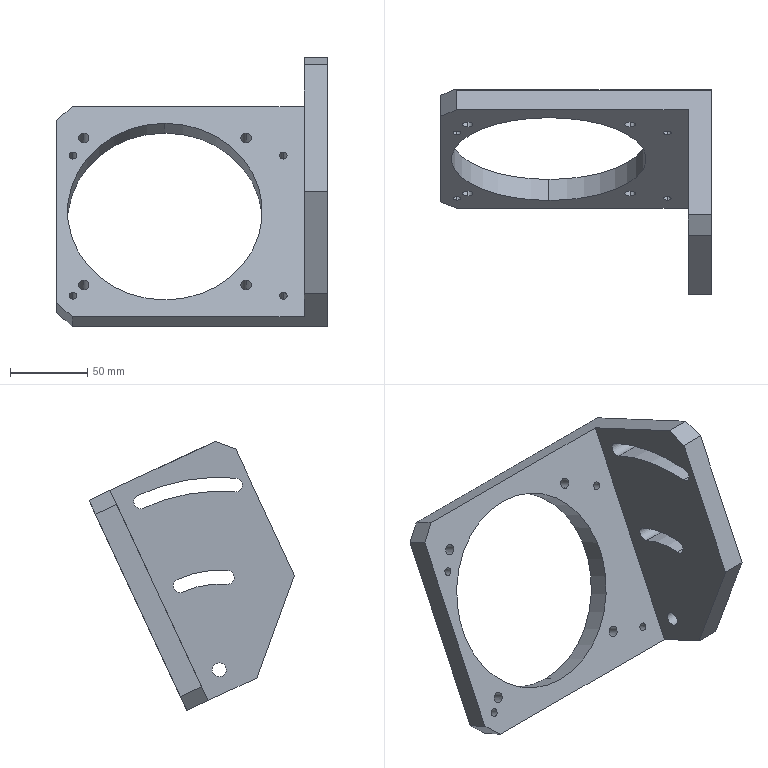Component | SolidWorks | 17081801-804-004A-1 | 1 solid | 41 faces | box 175 x 132.47 x 173.98 mm | volume 357939 mm3 | cylinder 28 | plane 13 | commonest cylinder face diameters 5 x8 6.8 x8 9 x6 126 x2 111 x1 129 x1 231 x1 249 x1 | material AL6061
build123d program:
from build123d import *

# Parameters (mm, degrees)
BOSS_EXTRUDE2_DEPTH   = 75
SKETCH17_R            = 63
CUT_EXTRUDE2_DEPTH    = 197.087
M8_TAPPED_HOLE1_D     = 6.8
M8_TAPPED_HOLE1_DEPTH = 19.75
M8_TAPPED_HOLE1_TIP   = 2.043
M8_CLEARANCE_HOLE1_D  = 9
CUT_EXTRUDE1_DEPTH    = 209.507
CHAMFER2_SIZE         = 10
CHAMFER3_SIZE         = 50
M6_TAPPED_HOLE1_D     = 5
CHAMFER1_SIZE         = 1


with BuildPart() as part:
    # Sketch3 → Boss-Extrude2 (new, symmetric)
    with BuildSketch(Plane.XY):
        Polygon((-15, 15), (85, 15), (85, 0), (0, 0), (0, -160), (-15, -160), align=None)
    extrude(amount=BOSS_EXTRUDE2_DEPTH, both=True)

    # Sketch17 → Cut-Extrude2 (cut, through all)
    with BuildSketch(Plane(origin=(0, 0, 0), x_dir=(0, 0, -1), z_dir=(1, 0, 0))):
        with Locations((0, -90)):
            Circle(SKETCH17_R)
    extrude(amount=-CUT_EXTRUDE2_DEPTH, mode=Mode.SUBTRACT)

    # M8 Tapped Hole1
    with Locations(Plane(origin=(0, 0, 0), x_dir=(0, 0, -1), z_dir=(1, 0, 0))):
        with Locations((52.5, -37.5), (-52.5, -37.5), (-52.5, -142.5), (52.5, -142.5)):
            Hole(M8_TAPPED_HOLE1_D / 2, depth=M8_TAPPED_HOLE1_DEPTH)
            with Locations((0, 0, -(M8_TAPPED_HOLE1_DEPTH + M8_TAPPED_HOLE1_TIP / 2))):  # 118° drill point
                Cone(0, M8_TAPPED_HOLE1_D / 2, M8_TAPPED_HOLE1_TIP, mode=Mode.SUBTRACT)

    # M8 Clearance Hole1 (through all)
    with Locations(Plane(origin=(0, 15, 0), x_dir=(1, 0, 0), z_dir=(0, 1, 0))):
        with Locations((15, 60), (15, 0), (15, -60)):
            Hole(M8_CLEARANCE_HOLE1_D / 2)

    # Sketch16 → Cut-Extrude1 (cut, through all)
    with BuildSketch(Plane(origin=(0, 15, 0), x_dir=(1, 0, 0), z_dir=(0, 1, 0))):
        with BuildLine():
            ThreePointArc((15, -4.5), (31.694, -2.302), (47.25, 4.141))
            ThreePointArc((47.25, 4.141), (48.897, 10.288), (42.75, 11.936))
            ThreePointArc((42.75, 11.936), (29.364, 6.391), (15, 4.5))
            ThreePointArc((15, 4.5), (10.5, 0), (15, -4.5))
        make_face()
        with BuildLine():
            ThreePointArc((15, -64.5), (47.223, -60.258), (77.25, -47.82))
            ThreePointArc((77.25, -47.82), (78.897, -41.673), (72.75, -40.026))
            ThreePointArc((72.75, -40.026), (44.894, -51.564), (15, -55.5))
            ThreePointArc((15, -55.5), (10.5, -60), (15, -64.5))
        make_face()
    extrude(amount=-CUT_EXTRUDE1_DEPTH, mode=Mode.SUBTRACT)

    # Chamfer2
    chamfer2_edges = [part.edges().sort_by_distance(p)[0] for p in [
        (85, 7.5, 75),
        (-7.5, -160, 75),
        (-7.5, -160, -75),
    ]]
    chamfer(chamfer2_edges, length=CHAMFER2_SIZE)

    # Chamfer3
    chamfer3_edges = [part.edges().sort_by_distance(p)[0] for p in [
        (85, 7.5, -75),
    ]]
    chamfer(chamfer3_edges, length=CHAMFER3_SIZE)

    # M6 Tapped Hole1 (through all)
    with Locations(Plane.ZY.offset(15)):
        with Locations((40, -149.5), (40, -13.5), (-60, -149.5), (-60, -13.5)):
            Hole(M6_TAPPED_HOLE1_D / 2)

    # Chamfer1
    chamfer1_edges = [part.edges().sort_by_distance(p)[0] for p in [
        (-15, -67.5, 75),
    ]]
    chamfer(chamfer1_edges, length=CHAMFER1_SIZE)


solid = part.part

# Placed as in the assembly
solid = solid.moved(Location((-141.5, 2173.352, 239.039), (-25, 0, -90)))